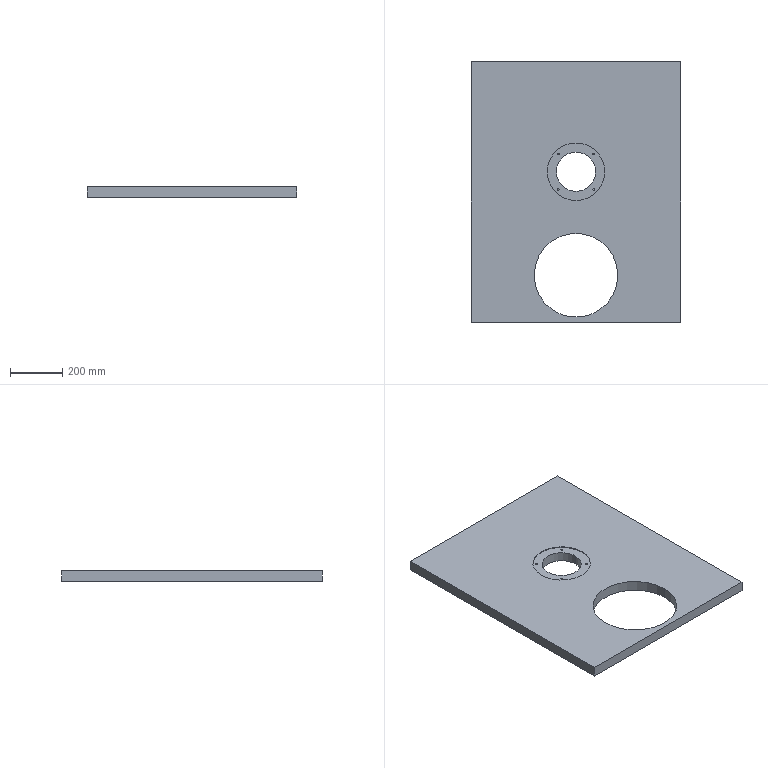Component | SolidWorks | JF21-80.1-1-3(_)-1-SOLID74-1 | 1 solid | 33 faces | box 800 x 995 x 40 mm | volume 27850861 mm3 | cylinder 16 | cone 10 | plane 7 | commonest cylinder face diameters 6.8 x8 8.5 x2 220 x2 320 x2 150 x2
STEP:
#1=COLOUR_RGB('',0.7922,0.8196,0.9333);
#2=FILL_AREA_STYLE_COLOUR('',#1);
#3=FILL_AREA_STYLE('',(#2));
#4=SURFACE_STYLE_FILL_AREA(#3);
#5=SURFACE_SIDE_STYLE('',(#4));
#6=SURFACE_STYLE_USAGE(.BOTH.,#5);
#7=PRESENTATION_STYLE_ASSIGNMENT((#6));
#8=CARTESIAN_POINT('',(0.,15.669,25.226));
#9=VERTEX_POINT('',#8);
#10=CARTESIAN_POINT('',(0.,15.669,25.561));
#11=VERTEX_POINT('',#10);
#12=CARTESIAN_POINT('',(0.,15.669,25.394));
#13=DIRECTION('',(0.,1.,0.));
#14=DIRECTION('',(0.,0.,1.));
#15=AXIS2_PLACEMENT_3D('',#12,#13,#14);
#16=CIRCLE('',#15,0.1673);
#17=EDGE_CURVE('',#9,#11,#16,.T.);
#18=ORIENTED_EDGE('',*,*,#17,.F.);
#19=CARTESIAN_POINT('',(0.,16.535,25.226));
#20=VERTEX_POINT('',#19);
#21=CARTESIAN_POINT('',(0.,16.535,25.226));
#22=DIRECTION('',(0.,1.,0.));
#23=VECTOR('',#22,39.37);
#24=LINE('',#21,#23);
#25=EDGE_CURVE('',#9,#20,#24,.T.);
#26=ORIENTED_EDGE('',*,*,#25,.T.);
#27=CARTESIAN_POINT('',(0.,16.535,25.561));
#28=VERTEX_POINT('',#27);
#29=CARTESIAN_POINT('',(0.,16.535,25.394));
#30=DIRECTION('',(0.,1.,0.));
#31=DIRECTION('',(0.,0.,1.));
#32=AXIS2_PLACEMENT_3D('',#29,#30,#31);
#33=CIRCLE('',#32,0.1673);
#34=EDGE_CURVE('',#20,#28,#33,.T.);
#35=ORIENTED_EDGE('',*,*,#34,.T.);
#36=CARTESIAN_POINT('',(0.,16.535,25.561));
#37=DIRECTION('',(0.,1.,0.));
#38=VECTOR('',#37,39.37);
#39=LINE('',#36,#38);
#40=EDGE_CURVE('',#11,#28,#39,.T.);
#41=ORIENTED_EDGE('',*,*,#40,.F.);
#42=EDGE_LOOP('',(#18,#26,#35,#41));
#43=FACE_OUTER_BOUND('',#42,.T.);
#44=CARTESIAN_POINT('',(0.,16.535,25.394));
#45=DIRECTION('',(0.,1.,0.));
#46=DIRECTION('',(0.,0.,-1.));
#47=AXIS2_PLACEMENT_3D('',#44,#45,#46);
#48=CYLINDRICAL_SURFACE('',#47,0.1673);
#49=ADVANCED_FACE('',(#43),#48,.F.);
#50=CARTESIAN_POINT('',(-0.,15.569,25.394));
#51=VERTEX_POINT('',#50);
#52=CARTESIAN_POINT('',(0.,15.669,25.561));
#53=DIRECTION('',(0.,0.515,0.8572));
#54=VECTOR('',#53,39.37);
#55=LINE('',#52,#54);
#56=EDGE_CURVE('',#51,#11,#55,.T.);
#57=ORIENTED_EDGE('',*,*,#56,.F.);
#58=CARTESIAN_POINT('',(0.,15.669,25.226));
#59=DIRECTION('',(0.,0.515,-0.8572));
#60=VECTOR('',#59,39.37);
#61=LINE('',#58,#60);
#62=EDGE_CURVE('',#51,#9,#61,.T.);
#63=ORIENTED_EDGE('',*,*,#62,.T.);
#64=ORIENTED_EDGE('',*,*,#17,.T.);
#65=EDGE_LOOP('',(#57,#63,#64));
#66=FACE_OUTER_BOUND('',#65,.T.);
#67=CARTESIAN_POINT('',(0.,15.669,25.394));
#68=DIRECTION('',(0.,1.,0.));
#69=DIRECTION('',(0.,0.,-1.));
#70=AXIS2_PLACEMENT_3D('',#67,#68,#69);
#71=CONICAL_SURFACE('',#70,0.1673,1.03);
#72=ADVANCED_FACE('',(#66),#71,.F.);
#73=CARTESIAN_POINT('',(2.539,-2.673,25.679));
#74=VERTEX_POINT('',#73);
#75=CARTESIAN_POINT('',(2.806,-2.673,25.679));
#76=VERTEX_POINT('',#75);
#77=CARTESIAN_POINT('',(2.673,-2.673,25.679));
#78=DIRECTION('',(0.,0.,1.));
#79=DIRECTION('',(1.,0.,0.));
#80=AXIS2_PLACEMENT_3D('',#77,#78,#79);
#81=CIRCLE('',#80,0.1339);
#82=EDGE_CURVE('',#74,#76,#81,.T.);
#83=ORIENTED_EDGE('',*,*,#82,.F.);
#84=CARTESIAN_POINT('',(2.539,-2.673,26.457));
#85=VERTEX_POINT('',#84);
#86=CARTESIAN_POINT('',(2.539,-2.673,26.457));
#87=DIRECTION('',(0.,0.,1.));
#88=VECTOR('',#87,39.37);
#89=LINE('',#86,#88);
#90=EDGE_CURVE('',#74,#85,#89,.T.);
#91=ORIENTED_EDGE('',*,*,#90,.T.);
#92=CARTESIAN_POINT('',(2.806,-2.673,26.457));
#93=VERTEX_POINT('',#92);
#94=CARTESIAN_POINT('',(2.673,-2.673,26.457));
#95=DIRECTION('',(0.,0.,1.));
#96=DIRECTION('',(1.,0.,0.));
#97=AXIS2_PLACEMENT_3D('',#94,#95,#96);
#98=CIRCLE('',#97,0.1339);
#99=EDGE_CURVE('',#85,#93,#98,.T.);
#100=ORIENTED_EDGE('',*,*,#99,.T.);
#101=CARTESIAN_POINT('',(2.806,-2.673,26.457));
#102=DIRECTION('',(0.,0.,1.));
#103=VECTOR('',#102,39.37);
#104=LINE('',#101,#103);
#105=EDGE_CURVE('',#76,#93,#104,.T.);
#106=ORIENTED_EDGE('',*,*,#105,.F.);
#107=EDGE_LOOP('',(#83,#91,#100,#106));
#108=FACE_OUTER_BOUND('',#107,.T.);
#109=CARTESIAN_POINT('',(2.673,-2.673,26.457));
#110=DIRECTION('',(0.,0.,1.));
#111=DIRECTION('',(-1.,0.,0.));
#112=AXIS2_PLACEMENT_3D('',#109,#110,#111);
#113=CYLINDRICAL_SURFACE('',#112,0.1339);
#114=ADVANCED_FACE('',(#108),#113,.F.);
#115=CARTESIAN_POINT('',(2.673,-2.673,25.599));
#116=VERTEX_POINT('',#115);
#117=CARTESIAN_POINT('',(2.806,-2.673,25.679));
#118=DIRECTION('',(0.8572,0.,0.515));
#119=VECTOR('',#118,39.37);
#120=LINE('',#117,#119);
#121=EDGE_CURVE('',#116,#76,#120,.T.);
#122=ORIENTED_EDGE('',*,*,#121,.F.);
#123=CARTESIAN_POINT('',(2.539,-2.673,25.679));
#124=DIRECTION('',(-0.8572,0.,0.515));
#125=VECTOR('',#124,39.37);
#126=LINE('',#123,#125);
#127=EDGE_CURVE('',#116,#74,#126,.T.);
#128=ORIENTED_EDGE('',*,*,#127,.T.);
#129=ORIENTED_EDGE('',*,*,#82,.T.);
#130=EDGE_LOOP('',(#122,#128,#129));
#131=FACE_OUTER_BOUND('',#130,.T.);
#132=CARTESIAN_POINT('',(2.673,-2.673,25.679));
#133=DIRECTION('',(0.,0.,1.));
#134=DIRECTION('',(-1.,0.,0.));
#135=AXIS2_PLACEMENT_3D('',#132,#133,#134);
#136=CONICAL_SURFACE('',#135,0.1339,1.03);
#137=ADVANCED_FACE('',(#131),#136,.F.);
#138=CARTESIAN_POINT('',(-2.806,-2.673,25.679));
#139=VERTEX_POINT('',#138);
#140=CARTESIAN_POINT('',(-2.539,-2.673,25.679));
#141=VERTEX_POINT('',#140);
#142=CARTESIAN_POINT('',(-2.673,-2.673,25.679));
#143=DIRECTION('',(0.,0.,1.));
#144=DIRECTION('',(1.,0.,0.));
#145=AXIS2_PLACEMENT_3D('',#142,#143,#144);
#146=CIRCLE('',#145,0.1339);
#147=EDGE_CURVE('',#139,#141,#146,.T.);
#148=ORIENTED_EDGE('',*,*,#147,.F.);
#149=CARTESIAN_POINT('',(-2.806,-2.673,26.457));
#150=VERTEX_POINT('',#149);
#151=CARTESIAN_POINT('',(-2.806,-2.673,26.457));
#152=DIRECTION('',(0.,0.,1.));
#153=VECTOR('',#152,39.37);
#154=LINE('',#151,#153);
#155=EDGE_CURVE('',#139,#150,#154,.T.);
#156=ORIENTED_EDGE('',*,*,#155,.T.);
#157=CARTESIAN_POINT('',(-2.539,-2.673,26.457));
#158=VERTEX_POINT('',#157);
#159=CARTESIAN_POINT('',(-2.673,-2.673,26.457));
#160=DIRECTION('',(0.,0.,1.));
#161=DIRECTION('',(1.,0.,0.));
#162=AXIS2_PLACEMENT_3D('',#159,#160,#161);
#163=CIRCLE('',#162,0.1339);
#164=EDGE_CURVE('',#150,#158,#163,.T.);
#165=ORIENTED_EDGE('',*,*,#164,.T.);
#166=CARTESIAN_POINT('',(-2.539,-2.673,26.457));
#167=DIRECTION('',(0.,0.,1.));
#168=VECTOR('',#167,39.37);
#169=LINE('',#166,#168);
#170=EDGE_CURVE('',#141,#158,#169,.T.);
#171=ORIENTED_EDGE('',*,*,#170,.F.);
#172=EDGE_LOOP('',(#148,#156,#165,#171));
#173=FACE_OUTER_BOUND('',#172,.T.);
#174=CARTESIAN_POINT('',(-2.673,-2.673,26.457));
#175=DIRECTION('',(0.,0.,1.));
#176=DIRECTION('',(-1.,0.,0.));
#177=AXIS2_PLACEMENT_3D('',#174,#175,#176);
#178=CYLINDRICAL_SURFACE('',#177,0.1339);
#179=ADVANCED_FACE('',(#173),#178,.F.);
#180=CARTESIAN_POINT('',(-2.673,-2.673,25.599));
#181=VERTEX_POINT('',#180);
#182=CARTESIAN_POINT('',(-2.539,-2.673,25.679));
#183=DIRECTION('',(0.8572,0.,0.515));
#184=VECTOR('',#183,39.37);
#185=LINE('',#182,#184);
#186=EDGE_CURVE('',#181,#141,#185,.T.);
#187=ORIENTED_EDGE('',*,*,#186,.F.);
#188=CARTESIAN_POINT('',(-2.806,-2.673,25.679));
#189=DIRECTION('',(-0.8572,0.,0.515));
#190=VECTOR('',#189,39.37);
#191=LINE('',#188,#190);
#192=EDGE_CURVE('',#181,#139,#191,.T.);
#193=ORIENTED_EDGE('',*,*,#192,.T.);
#194=ORIENTED_EDGE('',*,*,#147,.T.);
#195=EDGE_LOOP('',(#187,#193,#194));
#196=FACE_OUTER_BOUND('',#195,.T.);
#197=CARTESIAN_POINT('',(-2.673,-2.673,25.679));
#198=DIRECTION('',(0.,0.,1.));
#199=DIRECTION('',(-1.,0.,0.));
#200=AXIS2_PLACEMENT_3D('',#197,#198,#199);
#201=CONICAL_SURFACE('',#200,0.1339,1.03);
#202=ADVANCED_FACE('',(#196),#201,.F.);
#203=CARTESIAN_POINT('',(-2.806,2.673,25.679));
#204=VERTEX_POINT('',#203);
#205=CARTESIAN_POINT('',(-2.539,2.673,25.679));
#206=VERTEX_POINT('',#205);
#207=CARTESIAN_POINT('',(-2.673,2.673,25.679));
#208=DIRECTION('',(0.,0.,1.));
#209=DIRECTION('',(1.,0.,0.));
#210=AXIS2_PLACEMENT_3D('',#207,#208,#209);
#211=CIRCLE('',#210,0.1339);
#212=EDGE_CURVE('',#204,#206,#211,.T.);
#213=ORIENTED_EDGE('',*,*,#212,.F.);
#214=CARTESIAN_POINT('',(-2.806,2.673,26.457));
#215=VERTEX_POINT('',#214);
#216=CARTESIAN_POINT('',(-2.806,2.673,26.457));
#217=DIRECTION('',(0.,0.,1.));
#218=VECTOR('',#217,39.37);
#219=LINE('',#216,#218);
#220=EDGE_CURVE('',#204,#215,#219,.T.);
#221=ORIENTED_EDGE('',*,*,#220,.T.);
#222=CARTESIAN_POINT('',(-2.539,2.673,26.457));
#223=VERTEX_POINT('',#222);
#224=CARTESIAN_POINT('',(-2.673,2.673,26.457));
#225=DIRECTION('',(0.,0.,1.));
#226=DIRECTION('',(1.,0.,0.));
#227=AXIS2_PLACEMENT_3D('',#224,#225,#226);
#228=CIRCLE('',#227,0.1339);
#229=EDGE_CURVE('',#215,#223,#228,.T.);
#230=ORIENTED_EDGE('',*,*,#229,.T.);
#231=CARTESIAN_POINT('',(-2.539,2.673,26.457));
#232=DIRECTION('',(0.,0.,1.));
#233=VECTOR('',#232,39.37);
#234=LINE('',#231,#233);
#235=EDGE_CURVE('',#206,#223,#234,.T.);
#236=ORIENTED_EDGE('',*,*,#235,.F.);
#237=EDGE_LOOP('',(#213,#221,#230,#236));
#238=FACE_OUTER_BOUND('',#237,.T.);
#239=CARTESIAN_POINT('',(-2.673,2.673,26.457));
#240=DIRECTION('',(0.,0.,1.));
#241=DIRECTION('',(-1.,0.,0.));
#242=AXIS2_PLACEMENT_3D('',#239,#240,#241);
#243=CYLINDRICAL_SURFACE('',#242,0.1339);
#244=ADVANCED_FACE('',(#238),#243,.F.);
#245=CARTESIAN_POINT('',(-2.673,2.673,25.599));
#246=VERTEX_POINT('',#245);
#247=CARTESIAN_POINT('',(-2.539,2.673,25.679));
#248=DIRECTION('',(0.8572,0.,0.515));
#249=VECTOR('',#248,39.37);
#250=LINE('',#247,#249);
#251=EDGE_CURVE('',#246,#206,#250,.T.);
#252=ORIENTED_EDGE('',*,*,#251,.F.);
#253=CARTESIAN_POINT('',(-2.806,2.673,25.679));
#254=DIRECTION('',(-0.8572,0.,0.515));
#255=VECTOR('',#254,39.37);
#256=LINE('',#253,#255);
#257=EDGE_CURVE('',#246,#204,#256,.T.);
#258=ORIENTED_EDGE('',*,*,#257,.T.);
#259=ORIENTED_EDGE('',*,*,#212,.T.);
#260=EDGE_LOOP('',(#252,#258,#259));
#261=FACE_OUTER_BOUND('',#260,.T.);
#262=CARTESIAN_POINT('',(-2.673,2.673,25.679));
#263=DIRECTION('',(0.,0.,1.));
#264=DIRECTION('',(-1.,0.,0.));
#265=AXIS2_PLACEMENT_3D('',#262,#263,#264);
#266=CONICAL_SURFACE('',#265,0.1339,1.03);
#267=ADVANCED_FACE('',(#261),#266,.F.);
#268=CARTESIAN_POINT('',(2.539,2.673,25.679));
#269=VERTEX_POINT('',#268);
#270=CARTESIAN_POINT('',(2.806,2.673,25.679));
#271=VERTEX_POINT('',#270);
#272=CARTESIAN_POINT('',(2.673,2.673,25.679));
#273=DIRECTION('',(0.,0.,1.));
#274=DIRECTION('',(1.,0.,0.));
#275=AXIS2_PLACEMENT_3D('',#272,#273,#274);
#276=CIRCLE('',#275,0.1339);
#277=EDGE_CURVE('',#269,#271,#276,.T.);
#278=ORIENTED_EDGE('',*,*,#277,.F.);
#279=CARTESIAN_POINT('',(2.539,2.673,26.457));
#280=VERTEX_POINT('',#279);
#281=CARTESIAN_POINT('',(2.539,2.673,26.457));
#282=DIRECTION('',(0.,0.,1.));
#283=VECTOR('',#282,39.37);
#284=LINE('',#281,#283);
#285=EDGE_CURVE('',#269,#280,#284,.T.);
#286=ORIENTED_EDGE('',*,*,#285,.T.);
#287=CARTESIAN_POINT('',(2.806,2.673,26.457));
#288=VERTEX_POINT('',#287);
#289=CARTESIAN_POINT('',(2.673,2.673,26.457));
#290=DIRECTION('',(0.,0.,1.));
#291=DIRECTION('',(1.,0.,0.));
#292=AXIS2_PLACEMENT_3D('',#289,#290,#291);
#293=CIRCLE('',#292,0.1339);
#294=EDGE_CURVE('',#280,#288,#293,.T.);
#295=ORIENTED_EDGE('',*,*,#294,.T.);
#296=CARTESIAN_POINT('',(2.806,2.673,26.457));
#297=DIRECTION('',(0.,0.,1.));
#298=VECTOR('',#297,39.37);
#299=LINE('',#296,#298);
#300=EDGE_CURVE('',#271,#288,#299,.T.);
#301=ORIENTED_EDGE('',*,*,#300,.F.);
#302=EDGE_LOOP('',(#278,#286,#295,#301));
#303=FACE_OUTER_BOUND('',#302,.T.);
#304=CARTESIAN_POINT('',(2.673,2.673,26.457));
#305=DIRECTION('',(0.,0.,1.));
#306=DIRECTION('',(-1.,0.,0.));
#307=AXIS2_PLACEMENT_3D('',#304,#305,#306);
#308=CYLINDRICAL_SURFACE('',#307,0.1339);
#309=ADVANCED_FACE('',(#303),#308,.F.);
#310=CARTESIAN_POINT('',(2.673,2.673,25.599));
#311=VERTEX_POINT('',#310);
#312=CARTESIAN_POINT('',(2.806,2.673,25.679));
#313=DIRECTION('',(0.8572,0.,0.515));
#314=VECTOR('',#313,39.37);
#315=LINE('',#312,#314);
#316=EDGE_CURVE('',#311,#271,#315,.T.);
#317=ORIENTED_EDGE('',*,*,#316,.F.);
#318=CARTESIAN_POINT('',(2.539,2.673,25.679));
#319=DIRECTION('',(-0.8572,0.,0.515));
#320=VECTOR('',#319,39.37);
#321=LINE('',#318,#320);
#322=EDGE_CURVE('',#311,#269,#321,.T.);
#323=ORIENTED_EDGE('',*,*,#322,.T.);
#324=ORIENTED_EDGE('',*,*,#277,.T.);
#325=EDGE_LOOP('',(#317,#323,#324));
#326=FACE_OUTER_BOUND('',#325,.T.);
#327=CARTESIAN_POINT('',(2.673,2.673,25.679));
#328=DIRECTION('',(0.,0.,1.));
#329=DIRECTION('',(-1.,0.,0.));
#330=AXIS2_PLACEMENT_3D('',#327,#328,#329);
#331=CONICAL_SURFACE('',#330,0.1339,1.03);
#332=ADVANCED_FACE('',(#326),#331,.F.);
#333=CARTESIAN_POINT('',(-4.331,0.,26.457));
#334=VERTEX_POINT('',#333);
#335=CARTESIAN_POINT('',(4.331,0.,26.457));
#336=VERTEX_POINT('',#335);
#337=CARTESIAN_POINT('',(0.,0.,26.457));
#338=DIRECTION('',(0.,0.,1.));
#339=DIRECTION('',(1.,0.,0.));
#340=AXIS2_PLACEMENT_3D('',#337,#338,#339);
#341=CIRCLE('',#340,4.331);
#342=EDGE_CURVE('',#334,#336,#341,.T.);
#343=ORIENTED_EDGE('',*,*,#342,.F.);
#344=CARTESIAN_POINT('',(-4.331,0.,26.575));
#345=VERTEX_POINT('',#344);
#346=CARTESIAN_POINT('',(-4.331,0.,26.457));
#347=DIRECTION('',(0.,0.,1.));
#348=VECTOR('',#347,39.37);
#349=LINE('',#346,#348);
#350=EDGE_CURVE('',#334,#345,#349,.T.);
#351=ORIENTED_EDGE('',*,*,#350,.T.);
#352=CARTESIAN_POINT('',(4.331,0.,26.575));
#353=VERTEX_POINT('',#352);
#354=CARTESIAN_POINT('',(0.,0.,26.575));
#355=DIRECTION('',(0.,0.,1.));
#356=DIRECTION('',(1.,0.,0.));
#357=AXIS2_PLACEMENT_3D('',#354,#355,#356);
#358=CIRCLE('',#357,4.331);
#359=EDGE_CURVE('',#345,#353,#358,.T.);
#360=ORIENTED_EDGE('',*,*,#359,.T.);
#361=CARTESIAN_POINT('',(4.331,0.,26.457));
#362=DIRECTION('',(0.,0.,1.));
#363=VECTOR('',#362,39.37);
#364=LINE('',#361,#363);
#365=EDGE_CURVE('',#336,#353,#364,.T.);
#366=ORIENTED_EDGE('',*,*,#365,.F.);
#367=EDGE_LOOP('',(#343,#351,#360,#366));
#368=FACE_OUTER_BOUND('',#367,.T.);
#369=CARTESIAN_POINT('',(0.,0.,26.457));
#370=DIRECTION('',(0.,0.,1.));
#371=DIRECTION('',(-1.,0.,0.));
#372=AXIS2_PLACEMENT_3D('',#369,#370,#371);
#373=CYLINDRICAL_SURFACE('',#372,4.331);
#374=ADVANCED_FACE('',(#368),#373,.F.);
#375=CARTESIAN_POINT('',(-6.299,-15.598,26.575));
#376=VERTEX_POINT('',#375);
#377=CARTESIAN_POINT('',(6.299,-15.598,26.575));
#378=VERTEX_POINT('',#377);
#379=CARTESIAN_POINT('',(0.,-15.598,26.575));
#380=DIRECTION('',(0.,0.,1.));
#381=DIRECTION('',(1.,0.,0.));
#382=AXIS2_PLACEMENT_3D('',#379,#380,#381);
#383=CIRCLE('',#382,6.299);
#384=EDGE_CURVE('',#376,#378,#383,.T.);
#385=ORIENTED_EDGE('',*,*,#384,.T.);
#386=CARTESIAN_POINT('',(6.299,-15.598,25.));
#387=VERTEX_POINT('',#386);
#388=CARTESIAN_POINT('',(6.299,-15.598,26.575));
#389=DIRECTION('',(0.,0.,1.));
#390=VECTOR('',#389,39.37);
#391=LINE('',#388,#390);
#392=EDGE_CURVE('',#387,#378,#391,.T.);
#393=ORIENTED_EDGE('',*,*,#392,.F.);
#394=CARTESIAN_POINT('',(-6.299,-15.598,25.));
#395=VERTEX_POINT('',#394);
#396=CARTESIAN_POINT('',(0.,-15.598,25.));
#397=DIRECTION('',(0.,0.,1.));
#398=DIRECTION('',(1.,0.,0.));
#399=AXIS2_PLACEMENT_3D('',#396,#397,#398);
#400=CIRCLE('',#399,6.299);
#401=EDGE_CURVE('',#395,#387,#400,.T.);
#402=ORIENTED_EDGE('',*,*,#401,.F.);
#403=CARTESIAN_POINT('',(-6.299,-15.598,26.575));
#404=DIRECTION('',(0.,0.,1.));
#405=VECTOR('',#404,39.37);
#406=LINE('',#403,#405);
#407=EDGE_CURVE('',#395,#376,#406,.T.);
#408=ORIENTED_EDGE('',*,*,#407,.T.);
#409=EDGE_LOOP('',(#385,#393,#402,#408));
#410=FACE_OUTER_BOUND('',#409,.T.);
#411=CARTESIAN_POINT('',(0.,-15.598,26.575));
#412=DIRECTION('',(0.,0.,-1.));
#413=DIRECTION('',(1.,0.,0.));
#414=AXIS2_PLACEMENT_3D('',#411,#412,#413);
#415=CYLINDRICAL_SURFACE('',#414,6.299);
#416=ADVANCED_FACE('',(#410),#415,.F.);
#417=CARTESIAN_POINT('',(-2.953,0.,26.457));
#418=VERTEX_POINT('',#417);
#419=CARTESIAN_POINT('',(2.953,0.,26.457));
#420=VERTEX_POINT('',#419);
#421=CARTESIAN_POINT('',(0.,0.,26.457));
#422=DIRECTION('',(0.,0.,1.));
#423=DIRECTION('',(1.,0.,0.));
#424=AXIS2_PLACEMENT_3D('',#421,#422,#423);
#425=CIRCLE('',#424,2.953);
#426=EDGE_CURVE('',#418,#420,#425,.T.);
#427=ORIENTED_EDGE('',*,*,#426,.T.);
#428=CARTESIAN_POINT('',(2.953,0.,25.));
#429=VERTEX_POINT('',#428);
#430=CARTESIAN_POINT('',(2.953,0.,26.575));
#431=DIRECTION('',(0.,0.,1.));
#432=VECTOR('',#431,39.37);
#433=LINE('',#430,#432);
#434=EDGE_CURVE('',#429,#420,#433,.T.);
#435=ORIENTED_EDGE('',*,*,#434,.F.);
#436=CARTESIAN_POINT('',(-2.953,0.,25.));
#437=VERTEX_POINT('',#436);
#438=CARTESIAN_POINT('',(0.,0.,25.));
#439=DIRECTION('',(0.,0.,1.));
#440=DIRECTION('',(1.,0.,0.));
#441=AXIS2_PLACEMENT_3D('',#438,#439,#440);
#442=CIRCLE('',#441,2.953);
#443=EDGE_CURVE('',#437,#429,#442,.T.);
#444=ORIENTED_EDGE('',*,*,#443,.F.);
#445=CARTESIAN_POINT('',(-2.953,0.,26.575));
#446=DIRECTION('',(0.,0.,1.));
#447=VECTOR('',#446,39.37);
#448=LINE('',#445,#447);
#449=EDGE_CURVE('',#437,#418,#448,.T.);
#450=ORIENTED_EDGE('',*,*,#449,.T.);
#451=EDGE_LOOP('',(#427,#435,#444,#450));
#452=FACE_OUTER_BOUND('',#451,.T.);
#453=CARTESIAN_POINT('',(0.,0.,26.575));
#454=DIRECTION('',(0.,0.,-1.));
#455=DIRECTION('',(1.,0.,0.));
#456=AXIS2_PLACEMENT_3D('',#453,#454,#455);
#457=CYLINDRICAL_SURFACE('',#456,2.953);
#458=ADVANCED_FACE('',(#452),#457,.F.);
#459=ORIENTED_EDGE('',*,*,#434,.T.);
#460=CARTESIAN_POINT('',(0.,0.,26.457));
#461=DIRECTION('',(0.,0.,1.));
#462=DIRECTION('',(1.,0.,0.));
#463=AXIS2_PLACEMENT_3D('',#460,#461,#462);
#464=CIRCLE('',#463,2.953);
#465=EDGE_CURVE('',#420,#418,#464,.T.);
#466=ORIENTED_EDGE('',*,*,#465,.T.);
#467=ORIENTED_EDGE('',*,*,#449,.F.);
#468=CARTESIAN_POINT('',(0.,0.,25.));
#469=DIRECTION('',(0.,0.,1.));
#470=DIRECTION('',(1.,0.,0.));
#471=AXIS2_PLACEMENT_3D('',#468,#469,#470);
#472=CIRCLE('',#471,2.953);
#473=EDGE_CURVE('',#429,#437,#472,.T.);
#474=ORIENTED_EDGE('',*,*,#473,.F.);
#475=EDGE_LOOP('',(#459,#466,#467,#474));
#476=FACE_OUTER_BOUND('',#475,.T.);
#477=CARTESIAN_POINT('',(0.,0.,26.575));
#478=DIRECTION('',(0.,0.,-1.));
#479=DIRECTION('',(1.,0.,0.));
#480=AXIS2_PLACEMENT_3D('',#477,#478,#479);
#481=CYLINDRICAL_SURFACE('',#480,2.953);
#482=ADVANCED_FACE('',(#476),#481,.F.);
#483=CARTESIAN_POINT('',(0.,0.,26.575));
#484=DIRECTION('',(0.,0.,1.));
#485=DIRECTION('',(1.,0.,0.));
#486=AXIS2_PLACEMENT_3D('',#483,#484,#485);
#487=CIRCLE('',#486,4.331);
#488=EDGE_CURVE('',#353,#345,#487,.T.);
#489=ORIENTED_EDGE('',*,*,#488,.F.);
#490=ORIENTED_EDGE('',*,*,#359,.F.);
#491=EDGE_LOOP('',(#489,#490));
#492=FACE_BOUND('',#491,.T.);
#493=ORIENTED_EDGE('',*,*,#384,.F.);
#494=CARTESIAN_POINT('',(0.,-15.598,26.575));
#495=DIRECTION('',(0.,0.,1.));
#496=DIRECTION('',(1.,0.,0.));
#497=AXIS2_PLACEMENT_3D('',#494,#495,#496);
#498=CIRCLE('',#497,6.299);
#499=EDGE_CURVE('',#378,#376,#498,.T.);
#500=ORIENTED_EDGE('',*,*,#499,.F.);
#501=EDGE_LOOP('',(#493,#500));
#502=FACE_BOUND('',#501,.T.);
#503=CARTESIAN_POINT('',(-15.748,16.535,26.575));
#504=VERTEX_POINT('',#503);
#505=CARTESIAN_POINT('',(-15.748,-22.638,26.575));
#506=VERTEX_POINT('',#505);
#507=CARTESIAN_POINT('',(-15.748,16.535,26.575));
#508=DIRECTION('',(0.,-1.,0.));
#509=VECTOR('',#508,39.37);
#510=LINE('',#507,#509);
#511=EDGE_CURVE('',#504,#506,#510,.T.);
#512=ORIENTED_EDGE('',*,*,#511,.T.);
#513=CARTESIAN_POINT('',(15.748,-22.638,26.575));
#514=VERTEX_POINT('',#513);
#515=CARTESIAN_POINT('',(-15.748,-22.638,26.575));
#516=DIRECTION('',(1.,0.,0.));
#517=VECTOR('',#516,39.37);
#518=LINE('',#515,#517);
#519=EDGE_CURVE('',#506,#514,#518,.T.);
#520=ORIENTED_EDGE('',*,*,#519,.T.);
#521=CARTESIAN_POINT('',(15.748,16.535,26.575));
#522=VERTEX_POINT('',#521);
#523=CARTESIAN_POINT('',(15.748,16.535,26.575));
#524=DIRECTION('',(0.,1.,0.));
#525=VECTOR('',#524,39.37);
#526=LINE('',#523,#525);
#527=EDGE_CURVE('',#514,#522,#526,.T.);
#528=ORIENTED_EDGE('',*,*,#527,.T.);
#529=CARTESIAN_POINT('',(-15.748,16.535,26.575));
#530=DIRECTION('',(-1.,0.,0.));
#531=VECTOR('',#530,39.37);
#532=LINE('',#529,#531);
#533=EDGE_CURVE('',#522,#504,#532,.T.);
#534=ORIENTED_EDGE('',*,*,#533,.T.);
#535=EDGE_LOOP('',(#512,#520,#528,#534));
#536=FACE_OUTER_BOUND('',#535,.T.);
#537=CARTESIAN_POINT('',(-15.748,-22.638,26.575));
#538=DIRECTION('',(0.,0.,1.));
#539=DIRECTION('',(-1.,0.,0.));
#540=AXIS2_PLACEMENT_3D('',#537,#538,#539);
#541=PLANE('',#540);
#542=ADVANCED_FACE('',(#492,#502,#536),#541,.T.);
#543=ORIENTED_EDGE('',*,*,#401,.T.);
#544=CARTESIAN_POINT('',(0.,-15.598,25.));
#545=DIRECTION('',(0.,0.,1.));
#546=DIRECTION('',(1.,0.,0.));
#547=AXIS2_PLACEMENT_3D('',#544,#545,#546);
#548=CIRCLE('',#547,6.299);
#549=EDGE_CURVE('',#387,#395,#548,.T.);
#550=ORIENTED_EDGE('',*,*,#549,.T.);
#551=EDGE_LOOP('',(#543,#550));
#552=FACE_BOUND('',#551,.T.);
#553=CARTESIAN_POINT('',(-15.748,16.535,25.));
#554=VERTEX_POINT('',#553);
#555=CARTESIAN_POINT('',(-15.748,-22.638,25.));
#556=VERTEX_POINT('',#555);
#557=CARTESIAN_POINT('',(-15.748,16.535,25.));
#558=DIRECTION('',(0.,-1.,0.));
#559=VECTOR('',#558,39.37);
#560=LINE('',#557,#559);
#561=EDGE_CURVE('',#554,#556,#560,.T.);
#562=ORIENTED_EDGE('',*,*,#561,.F.);
#563=CARTESIAN_POINT('',(15.748,16.535,25.));
#564=VERTEX_POINT('',#563);
#565=CARTESIAN_POINT('',(-15.748,16.535,25.));
#566=DIRECTION('',(-1.,0.,0.));
#567=VECTOR('',#566,39.37);
#568=LINE('',#565,#567);
#569=EDGE_CURVE('',#564,#554,#568,.T.);
#570=ORIENTED_EDGE('',*,*,#569,.F.);
#571=CARTESIAN_POINT('',(15.748,-22.638,25.));
#572=VERTEX_POINT('',#571);
#573=CARTESIAN_POINT('',(15.748,16.535,25.));
#574=DIRECTION('',(0.,1.,0.));
#575=VECTOR('',#574,39.37);
#576=LINE('',#573,#575);
#577=EDGE_CURVE('',#572,#564,#576,.T.);
#578=ORIENTED_EDGE('',*,*,#577,.F.);
#579=CARTESIAN_POINT('',(-15.748,-22.638,25.));
#580=DIRECTION('',(1.,0.,0.));
#581=VECTOR('',#580,39.37);
#582=LINE('',#579,#581);
#583=EDGE_CURVE('',#556,#572,#582,.T.);
#584=ORIENTED_EDGE('',*,*,#583,.F.);
#585=EDGE_LOOP('',(#562,#570,#578,#584));
#586=FACE_OUTER_BOUND('',#585,.T.);
#587=ORIENTED_EDGE('',*,*,#443,.T.);
#588=ORIENTED_EDGE('',*,*,#473,.T.);
#589=EDGE_LOOP('',(#587,#588));
#590=FACE_BOUND('',#589,.T.);
#591=CARTESIAN_POINT('',(-15.748,-22.638,25.));
#592=DIRECTION('',(0.,0.,1.));
#593=DIRECTION('',(-1.,0.,0.));
#594=AXIS2_PLACEMENT_3D('',#591,#592,#593);
#595=PLANE('',#594);
#596=ADVANCED_FACE('',(#552,#586,#590),#595,.F.);
#597=ORIENTED_EDGE('',*,*,#561,.T.);
#598=CARTESIAN_POINT('',(-15.748,-22.638,26.575));
#599=DIRECTION('',(0.,0.,-1.));
#600=VECTOR('',#599,39.37);
#601=LINE('',#598,#600);
#602=EDGE_CURVE('',#506,#556,#601,.T.);
#603=ORIENTED_EDGE('',*,*,#602,.F.);
#604=ORIENTED_EDGE('',*,*,#511,.F.);
#605=CARTESIAN_POINT('',(-15.748,16.535,26.575));
#606=DIRECTION('',(0.,0.,-1.));
#607=VECTOR('',#606,39.37);
#608=LINE('',#605,#607);
#609=EDGE_CURVE('',#504,#554,#608,.T.);
#610=ORIENTED_EDGE('',*,*,#609,.T.);
#611=EDGE_LOOP('',(#597,#603,#604,#610));
#612=FACE_OUTER_BOUND('',#611,.T.);
#613=CARTESIAN_POINT('',(-15.748,16.535,26.575));
#614=DIRECTION('',(1.,0.,0.));
#615=DIRECTION('',(0.,-1.,0.));
#616=AXIS2_PLACEMENT_3D('',#613,#614,#615);
#617=PLANE('',#616);
#618=ADVANCED_FACE('',(#612),#617,.F.);
#619=ORIENTED_EDGE('',*,*,#583,.T.);
#620=CARTESIAN_POINT('',(15.748,-22.638,26.575));
#621=DIRECTION('',(0.,0.,-1.));
#622=VECTOR('',#621,39.37);
#623=LINE('',#620,#622);
#624=EDGE_CURVE('',#514,#572,#623,.T.);
#625=ORIENTED_EDGE('',*,*,#624,.F.);
#626=ORIENTED_EDGE('',*,*,#519,.F.);
#627=ORIENTED_EDGE('',*,*,#602,.T.);
#628=EDGE_LOOP('',(#619,#625,#626,#627));
#629=FACE_OUTER_BOUND('',#628,.T.);
#630=CARTESIAN_POINT('',(-15.748,-22.638,26.575));
#631=DIRECTION('',(0.,1.,0.));
#632=DIRECTION('',(0.,0.,-1.));
#633=AXIS2_PLACEMENT_3D('',#630,#631,#632);
#634=PLANE('',#633);
#635=ADVANCED_FACE('',(#629),#634,.F.);
#636=ORIENTED_EDGE('',*,*,#577,.T.);
#637=CARTESIAN_POINT('',(15.748,16.535,26.575));
#638=DIRECTION('',(0.,0.,-1.));
#639=VECTOR('',#638,39.37);
#640=LINE('',#637,#639);
#641=EDGE_CURVE('',#522,#564,#640,.T.);
#642=ORIENTED_EDGE('',*,*,#641,.F.);
#643=ORIENTED_EDGE('',*,*,#527,.F.);
#644=ORIENTED_EDGE('',*,*,#624,.T.);
#645=EDGE_LOOP('',(#636,#642,#643,#644));
#646=FACE_OUTER_BOUND('',#645,.T.);
#647=CARTESIAN_POINT('',(15.748,16.535,26.575));
#648=DIRECTION('',(-1.,0.,0.));
#649=DIRECTION('',(0.,0.,-1.));
#650=AXIS2_PLACEMENT_3D('',#647,#648,#649);
#651=PLANE('',#650);
#652=ADVANCED_FACE('',(#646),#651,.F.);
#653=CARTESIAN_POINT('',(0.,16.535,25.394));
#654=DIRECTION('',(0.,1.,0.));
#655=DIRECTION('',(0.,0.,1.));
#656=AXIS2_PLACEMENT_3D('',#653,#654,#655);
#657=CIRCLE('',#656,0.1673);
#658=EDGE_CURVE('',#28,#20,#657,.T.);
#659=ORIENTED_EDGE('',*,*,#658,.F.);
#660=ORIENTED_EDGE('',*,*,#34,.F.);
#661=EDGE_LOOP('',(#659,#660));
#662=FACE_BOUND('',#661,.T.);
#663=ORIENTED_EDGE('',*,*,#569,.T.);
#664=ORIENTED_EDGE('',*,*,#609,.F.);
#665=ORIENTED_EDGE('',*,*,#533,.F.);
#666=ORIENTED_EDGE('',*,*,#641,.T.);
#667=EDGE_LOOP('',(#663,#664,#665,#666));
#668=FACE_OUTER_BOUND('',#667,.T.);
#669=CARTESIAN_POINT('',(-15.748,16.535,26.575));
#670=DIRECTION('',(0.,-1.,0.));
#671=DIRECTION('',(0.,0.,1.));
#672=AXIS2_PLACEMENT_3D('',#669,#670,#671);
#673=PLANE('',#672);
#674=ADVANCED_FACE('',(#662,#668),#673,.F.);
#675=ORIENTED_EDGE('',*,*,#392,.T.);
#676=ORIENTED_EDGE('',*,*,#499,.T.);
#677=ORIENTED_EDGE('',*,*,#407,.F.);
#678=ORIENTED_EDGE('',*,*,#549,.F.);
#679=EDGE_LOOP('',(#675,#676,#677,#678));
#680=FACE_OUTER_BOUND('',#679,.T.);
#681=CARTESIAN_POINT('',(0.,-15.598,26.575));
#682=DIRECTION('',(0.,0.,-1.));
#683=DIRECTION('',(1.,0.,0.));
#684=AXIS2_PLACEMENT_3D('',#681,#682,#683);
#685=CYLINDRICAL_SURFACE('',#684,6.299);
#686=ADVANCED_FACE('',(#680),#685,.F.);
#687=ORIENTED_EDGE('',*,*,#350,.F.);
#688=CARTESIAN_POINT('',(0.,0.,26.457));
#689=DIRECTION('',(0.,0.,1.));
#690=DIRECTION('',(1.,0.,0.));
#691=AXIS2_PLACEMENT_3D('',#688,#689,#690);
#692=CIRCLE('',#691,4.331);
#693=EDGE_CURVE('',#336,#334,#692,.T.);
#694=ORIENTED_EDGE('',*,*,#693,.F.);
#695=ORIENTED_EDGE('',*,*,#365,.T.);
#696=ORIENTED_EDGE('',*,*,#488,.T.);
#697=EDGE_LOOP('',(#687,#694,#695,#696));
#698=FACE_OUTER_BOUND('',#697,.T.);
#699=CARTESIAN_POINT('',(0.,0.,26.457));
#700=DIRECTION('',(0.,0.,1.));
#701=DIRECTION('',(-1.,0.,0.));
#702=AXIS2_PLACEMENT_3D('',#699,#700,#701);
#703=CYLINDRICAL_SURFACE('',#702,4.331);
#704=ADVANCED_FACE('',(#698),#703,.F.);
#705=CARTESIAN_POINT('',(2.673,-2.673,26.457));
#706=DIRECTION('',(0.,0.,1.));
#707=DIRECTION('',(1.,0.,0.));
#708=AXIS2_PLACEMENT_3D('',#705,#706,#707);
#709=CIRCLE('',#708,0.1339);
#710=EDGE_CURVE('',#93,#85,#709,.T.);
#711=ORIENTED_EDGE('',*,*,#710,.F.);
#712=ORIENTED_EDGE('',*,*,#99,.F.);
#713=EDGE_LOOP('',(#711,#712));
#714=FACE_BOUND('',#713,.T.);
#715=CARTESIAN_POINT('',(-2.673,-2.673,26.457));
#716=DIRECTION('',(0.,0.,1.));
#717=DIRECTION('',(1.,0.,0.));
#718=AXIS2_PLACEMENT_3D('',#715,#716,#717);
#719=CIRCLE('',#718,0.1339);
#720=EDGE_CURVE('',#158,#150,#719,.T.);
#721=ORIENTED_EDGE('',*,*,#720,.F.);
#722=ORIENTED_EDGE('',*,*,#164,.F.);
#723=EDGE_LOOP('',(#721,#722));
#724=FACE_BOUND('',#723,.T.);
#725=CARTESIAN_POINT('',(-2.673,2.673,26.457));
#726=DIRECTION('',(0.,0.,1.));
#727=DIRECTION('',(1.,0.,0.));
#728=AXIS2_PLACEMENT_3D('',#725,#726,#727);
#729=CIRCLE('',#728,0.1339);
#730=EDGE_CURVE('',#223,#215,#729,.T.);
#731=ORIENTED_EDGE('',*,*,#730,.F.);
#732=ORIENTED_EDGE('',*,*,#229,.F.);
#733=EDGE_LOOP('',(#731,#732));
#734=FACE_BOUND('',#733,.T.);
#735=CARTESIAN_POINT('',(2.673,2.673,26.457));
#736=DIRECTION('',(0.,0.,1.));
#737=DIRECTION('',(1.,0.,0.));
#738=AXIS2_PLACEMENT_3D('',#735,#736,#737);
#739=CIRCLE('',#738,0.1339);
#740=EDGE_CURVE('',#288,#280,#739,.T.);
#741=ORIENTED_EDGE('',*,*,#740,.F.);
#742=ORIENTED_EDGE('',*,*,#294,.F.);
#743=EDGE_LOOP('',(#741,#742));
#744=FACE_BOUND('',#743,.T.);
#745=ORIENTED_EDGE('',*,*,#426,.F.);
#746=ORIENTED_EDGE('',*,*,#465,.F.);
#747=EDGE_LOOP('',(#745,#746));
#748=FACE_BOUND('',#747,.T.);
#749=ORIENTED_EDGE('',*,*,#693,.T.);
#750=ORIENTED_EDGE('',*,*,#342,.T.);
#751=EDGE_LOOP('',(#749,#750));
#752=FACE_OUTER_BOUND('',#751,.T.);
#753=CARTESIAN_POINT('',(0.,0.,26.457));
#754=DIRECTION('',(0.,0.,1.));
#755=DIRECTION('',(-1.,0.,0.));
#756=AXIS2_PLACEMENT_3D('',#753,#754,#755);
#757=PLANE('',#756);
#758=ADVANCED_FACE('',(#714,#724,#734,#744,#748,#752),#757,.T.);
#759=ORIENTED_EDGE('',*,*,#322,.F.);
#760=ORIENTED_EDGE('',*,*,#316,.T.);
#761=CARTESIAN_POINT('',(2.673,2.673,25.679));
#762=DIRECTION('',(0.,0.,1.));
#763=DIRECTION('',(1.,0.,0.));
#764=AXIS2_PLACEMENT_3D('',#761,#762,#763);
#765=CIRCLE('',#764,0.1339);
#766=EDGE_CURVE('',#271,#269,#765,.T.);
#767=ORIENTED_EDGE('',*,*,#766,.T.);
#768=EDGE_LOOP('',(#759,#760,#767));
#769=FACE_OUTER_BOUND('',#768,.T.);
#770=CARTESIAN_POINT('',(2.673,2.673,25.679));
#771=DIRECTION('',(0.,0.,1.));
#772=DIRECTION('',(-1.,0.,0.));
#773=AXIS2_PLACEMENT_3D('',#770,#771,#772);
#774=CONICAL_SURFACE('',#773,0.1339,1.03);
#775=ADVANCED_FACE('',(#769),#774,.F.);
#776=ORIENTED_EDGE('',*,*,#285,.F.);
#777=ORIENTED_EDGE('',*,*,#766,.F.);
#778=ORIENTED_EDGE('',*,*,#300,.T.);
#779=ORIENTED_EDGE('',*,*,#740,.T.);
#780=EDGE_LOOP('',(#776,#777,#778,#779));
#781=FACE_OUTER_BOUND('',#780,.T.);
#782=CARTESIAN_POINT('',(2.673,2.673,26.457));
#783=DIRECTION('',(0.,0.,1.));
#784=DIRECTION('',(-1.,0.,0.));
#785=AXIS2_PLACEMENT_3D('',#782,#783,#784);
#786=CYLINDRICAL_SURFACE('',#785,0.1339);
#787=ADVANCED_FACE('',(#781),#786,.F.);
#788=ORIENTED_EDGE('',*,*,#257,.F.);
#789=ORIENTED_EDGE('',*,*,#251,.T.);
#790=CARTESIAN_POINT('',(-2.673,2.673,25.679));
#791=DIRECTION('',(0.,0.,1.));
#792=DIRECTION('',(1.,0.,0.));
#793=AXIS2_PLACEMENT_3D('',#790,#791,#792);
#794=CIRCLE('',#793,0.1339);
#795=EDGE_CURVE('',#206,#204,#794,.T.);
#796=ORIENTED_EDGE('',*,*,#795,.T.);
#797=EDGE_LOOP('',(#788,#789,#796));
#798=FACE_OUTER_BOUND('',#797,.T.);
#799=CARTESIAN_POINT('',(-2.673,2.673,25.679));
#800=DIRECTION('',(0.,0.,1.));
#801=DIRECTION('',(-1.,0.,0.));
#802=AXIS2_PLACEMENT_3D('',#799,#800,#801);
#803=CONICAL_SURFACE('',#802,0.1339,1.03);
#804=ADVANCED_FACE('',(#798),#803,.F.);
#805=ORIENTED_EDGE('',*,*,#220,.F.);
#806=ORIENTED_EDGE('',*,*,#795,.F.);
#807=ORIENTED_EDGE('',*,*,#235,.T.);
#808=ORIENTED_EDGE('',*,*,#730,.T.);
#809=EDGE_LOOP('',(#805,#806,#807,#808));
#810=FACE_OUTER_BOUND('',#809,.T.);
#811=CARTESIAN_POINT('',(-2.673,2.673,26.457));
#812=DIRECTION('',(0.,0.,1.));
#813=DIRECTION('',(-1.,0.,0.));
#814=AXIS2_PLACEMENT_3D('',#811,#812,#813);
#815=CYLINDRICAL_SURFACE('',#814,0.1339);
#816=ADVANCED_FACE('',(#810),#815,.F.);
#817=ORIENTED_EDGE('',*,*,#192,.F.);
#818=ORIENTED_EDGE('',*,*,#186,.T.);
#819=CARTESIAN_POINT('',(-2.673,-2.673,25.679));
#820=DIRECTION('',(0.,0.,1.));
#821=DIRECTION('',(1.,0.,0.));
#822=AXIS2_PLACEMENT_3D('',#819,#820,#821);
#823=CIRCLE('',#822,0.1339);
#824=EDGE_CURVE('',#141,#139,#823,.T.);
#825=ORIENTED_EDGE('',*,*,#824,.T.);
#826=EDGE_LOOP('',(#817,#818,#825));
#827=FACE_OUTER_BOUND('',#826,.T.);
#828=CARTESIAN_POINT('',(-2.673,-2.673,25.679));
#829=DIRECTION('',(0.,0.,1.));
#830=DIRECTION('',(-1.,0.,0.));
#831=AXIS2_PLACEMENT_3D('',#828,#829,#830);
#832=CONICAL_SURFACE('',#831,0.1339,1.03);
#833=ADVANCED_FACE('',(#827),#832,.F.);
#834=ORIENTED_EDGE('',*,*,#155,.F.);
#835=ORIENTED_EDGE('',*,*,#824,.F.);
#836=ORIENTED_EDGE('',*,*,#170,.T.);
#837=ORIENTED_EDGE('',*,*,#720,.T.);
#838=EDGE_LOOP('',(#834,#835,#836,#837));
#839=FACE_OUTER_BOUND('',#838,.T.);
#840=CARTESIAN_POINT('',(-2.673,-2.673,26.457));
#841=DIRECTION('',(0.,0.,1.));
#842=DIRECTION('',(-1.,0.,0.));
#843=AXIS2_PLACEMENT_3D('',#840,#841,#842);
#844=CYLINDRICAL_SURFACE('',#843,0.1339);
#845=ADVANCED_FACE('',(#839),#844,.F.);
#846=ORIENTED_EDGE('',*,*,#127,.F.);
#847=ORIENTED_EDGE('',*,*,#121,.T.);
#848=CARTESIAN_POINT('',(2.673,-2.673,25.679));
#849=DIRECTION('',(0.,0.,1.));
#850=DIRECTION('',(1.,0.,0.));
#851=AXIS2_PLACEMENT_3D('',#848,#849,#850);
#852=CIRCLE('',#851,0.1339);
#853=EDGE_CURVE('',#76,#74,#852,.T.);
#854=ORIENTED_EDGE('',*,*,#853,.T.);
#855=EDGE_LOOP('',(#846,#847,#854));
#856=FACE_OUTER_BOUND('',#855,.T.);
#857=CARTESIAN_POINT('',(2.673,-2.673,25.679));
#858=DIRECTION('',(0.,0.,1.));
#859=DIRECTION('',(-1.,0.,0.));
#860=AXIS2_PLACEMENT_3D('',#857,#858,#859);
#861=CONICAL_SURFACE('',#860,0.1339,1.03);
#862=ADVANCED_FACE('',(#856),#861,.F.);
#863=ORIENTED_EDGE('',*,*,#90,.F.);
#864=ORIENTED_EDGE('',*,*,#853,.F.);
#865=ORIENTED_EDGE('',*,*,#105,.T.);
#866=ORIENTED_EDGE('',*,*,#710,.T.);
#867=EDGE_LOOP('',(#863,#864,#865,#866));
#868=FACE_OUTER_BOUND('',#867,.T.);
#869=CARTESIAN_POINT('',(2.673,-2.673,26.457));
#870=DIRECTION('',(0.,0.,1.));
#871=DIRECTION('',(-1.,0.,0.));
#872=AXIS2_PLACEMENT_3D('',#869,#870,#871);
#873=CYLINDRICAL_SURFACE('',#872,0.1339);
#874=ADVANCED_FACE('',(#868),#873,.F.);
#875=ORIENTED_EDGE('',*,*,#62,.F.);
#876=ORIENTED_EDGE('',*,*,#56,.T.);
#877=CARTESIAN_POINT('',(0.,15.669,25.394));
#878=DIRECTION('',(0.,1.,0.));
#879=DIRECTION('',(0.,0.,1.));
#880=AXIS2_PLACEMENT_3D('',#877,#878,#879);
#881=CIRCLE('',#880,0.1673);
#882=EDGE_CURVE('',#11,#9,#881,.T.);
#883=ORIENTED_EDGE('',*,*,#882,.T.);
#884=EDGE_LOOP('',(#875,#876,#883));
#885=FACE_OUTER_BOUND('',#884,.T.);
#886=CARTESIAN_POINT('',(0.,15.669,25.394));
#887=DIRECTION('',(0.,1.,0.));
#888=DIRECTION('',(0.,0.,-1.));
#889=AXIS2_PLACEMENT_3D('',#886,#887,#888);
#890=CONICAL_SURFACE('',#889,0.1673,1.03);
#891=ADVANCED_FACE('',(#885),#890,.F.);
#892=ORIENTED_EDGE('',*,*,#25,.F.);
#893=ORIENTED_EDGE('',*,*,#882,.F.);
#894=ORIENTED_EDGE('',*,*,#40,.T.);
#895=ORIENTED_EDGE('',*,*,#658,.T.);
#896=EDGE_LOOP('',(#892,#893,#894,#895));
#897=FACE_OUTER_BOUND('',#896,.T.);
#898=CARTESIAN_POINT('',(0.,16.535,25.394));
#899=DIRECTION('',(0.,1.,0.));
#900=DIRECTION('',(0.,0.,-1.));
#901=AXIS2_PLACEMENT_3D('',#898,#899,#900);
#902=CYLINDRICAL_SURFACE('',#901,0.1673);
#903=ADVANCED_FACE('',(#897),#902,.F.);
#904=CLOSED_SHELL('',(#49,#72,#114,#137,#179,#202,#244,#267,#309,#332,#374,#416,#458,#482,#542,#596,#618,#635,#652,#674,#686,#704,#758,#775,#787,#804,#816,#833,#845,#862,#874,#891,#903));
#905=MANIFOLD_SOLID_BREP('',#904);
#906=STYLED_ITEM('',(#7),#905);
#907=(LENGTH_UNIT()NAMED_UNIT(*)SI_UNIT($,.METRE.));
#908=LENGTH_MEASURE_WITH_UNIT(LENGTH_MEASURE(0.0254),#907);
#909=DIMENSIONAL_EXPONENTS(1.,0.,0.,0.,0.,0.,0.);
#910=(CONVERSION_BASED_UNIT('',#908)LENGTH_UNIT()NAMED_UNIT(#909));
#911=UNCERTAINTY_MEASURE_WITH_UNIT(LENGTH_MEASURE(0.00001),#910,'','');
#912=(NAMED_UNIT(*)PLANE_ANGLE_UNIT()SI_UNIT($,.RADIAN.));
#913=(NAMED_UNIT(*)SI_UNIT($,.STERADIAN.)SOLID_ANGLE_UNIT());
#914=(GEOMETRIC_REPRESENTATION_CONTEXT(3)GLOBAL_UNCERTAINTY_ASSIGNED_CONTEXT((#911))GLOBAL_UNIT_ASSIGNED_CONTEXT((#910,#912,#913))REPRESENTATION_CONTEXT('',''));
#915=MECHANICAL_DESIGN_GEOMETRIC_PRESENTATION_REPRESENTATION('',(#906),#914);
#916=CARTESIAN_POINT('',(0.,0.,0.));
#917=DIRECTION('',(0.,0.,1.));
#918=DIRECTION('',(1.,0.,0.));
#919=AXIS2_PLACEMENT_3D('',#916,#917,#918);
#920=(LENGTH_UNIT()NAMED_UNIT(*)SI_UNIT($,.METRE.));
#921=LENGTH_MEASURE_WITH_UNIT(LENGTH_MEASURE(0.0254),#920);
#922=DIMENSIONAL_EXPONENTS(1.,0.,0.,0.,0.,0.,0.);
#923=(CONVERSION_BASED_UNIT('',#921)LENGTH_UNIT()NAMED_UNIT(#922));
#924=UNCERTAINTY_MEASURE_WITH_UNIT(LENGTH_MEASURE(0.00001),#923,'','');
#925=(NAMED_UNIT(*)PLANE_ANGLE_UNIT()SI_UNIT($,.RADIAN.));
#926=(NAMED_UNIT(*)SI_UNIT($,.STERADIAN.)SOLID_ANGLE_UNIT());
#927=(GEOMETRIC_REPRESENTATION_CONTEXT(3)GLOBAL_UNCERTAINTY_ASSIGNED_CONTEXT((#924))GLOBAL_UNIT_ASSIGNED_CONTEXT((#923,#925,#926))REPRESENTATION_CONTEXT('',''));
#928=ADVANCED_BREP_SHAPE_REPRESENTATION('',(#905,#919),#927);
#929=PRESENTATION_LAYER_ASSIGNMENT('','',(#906));